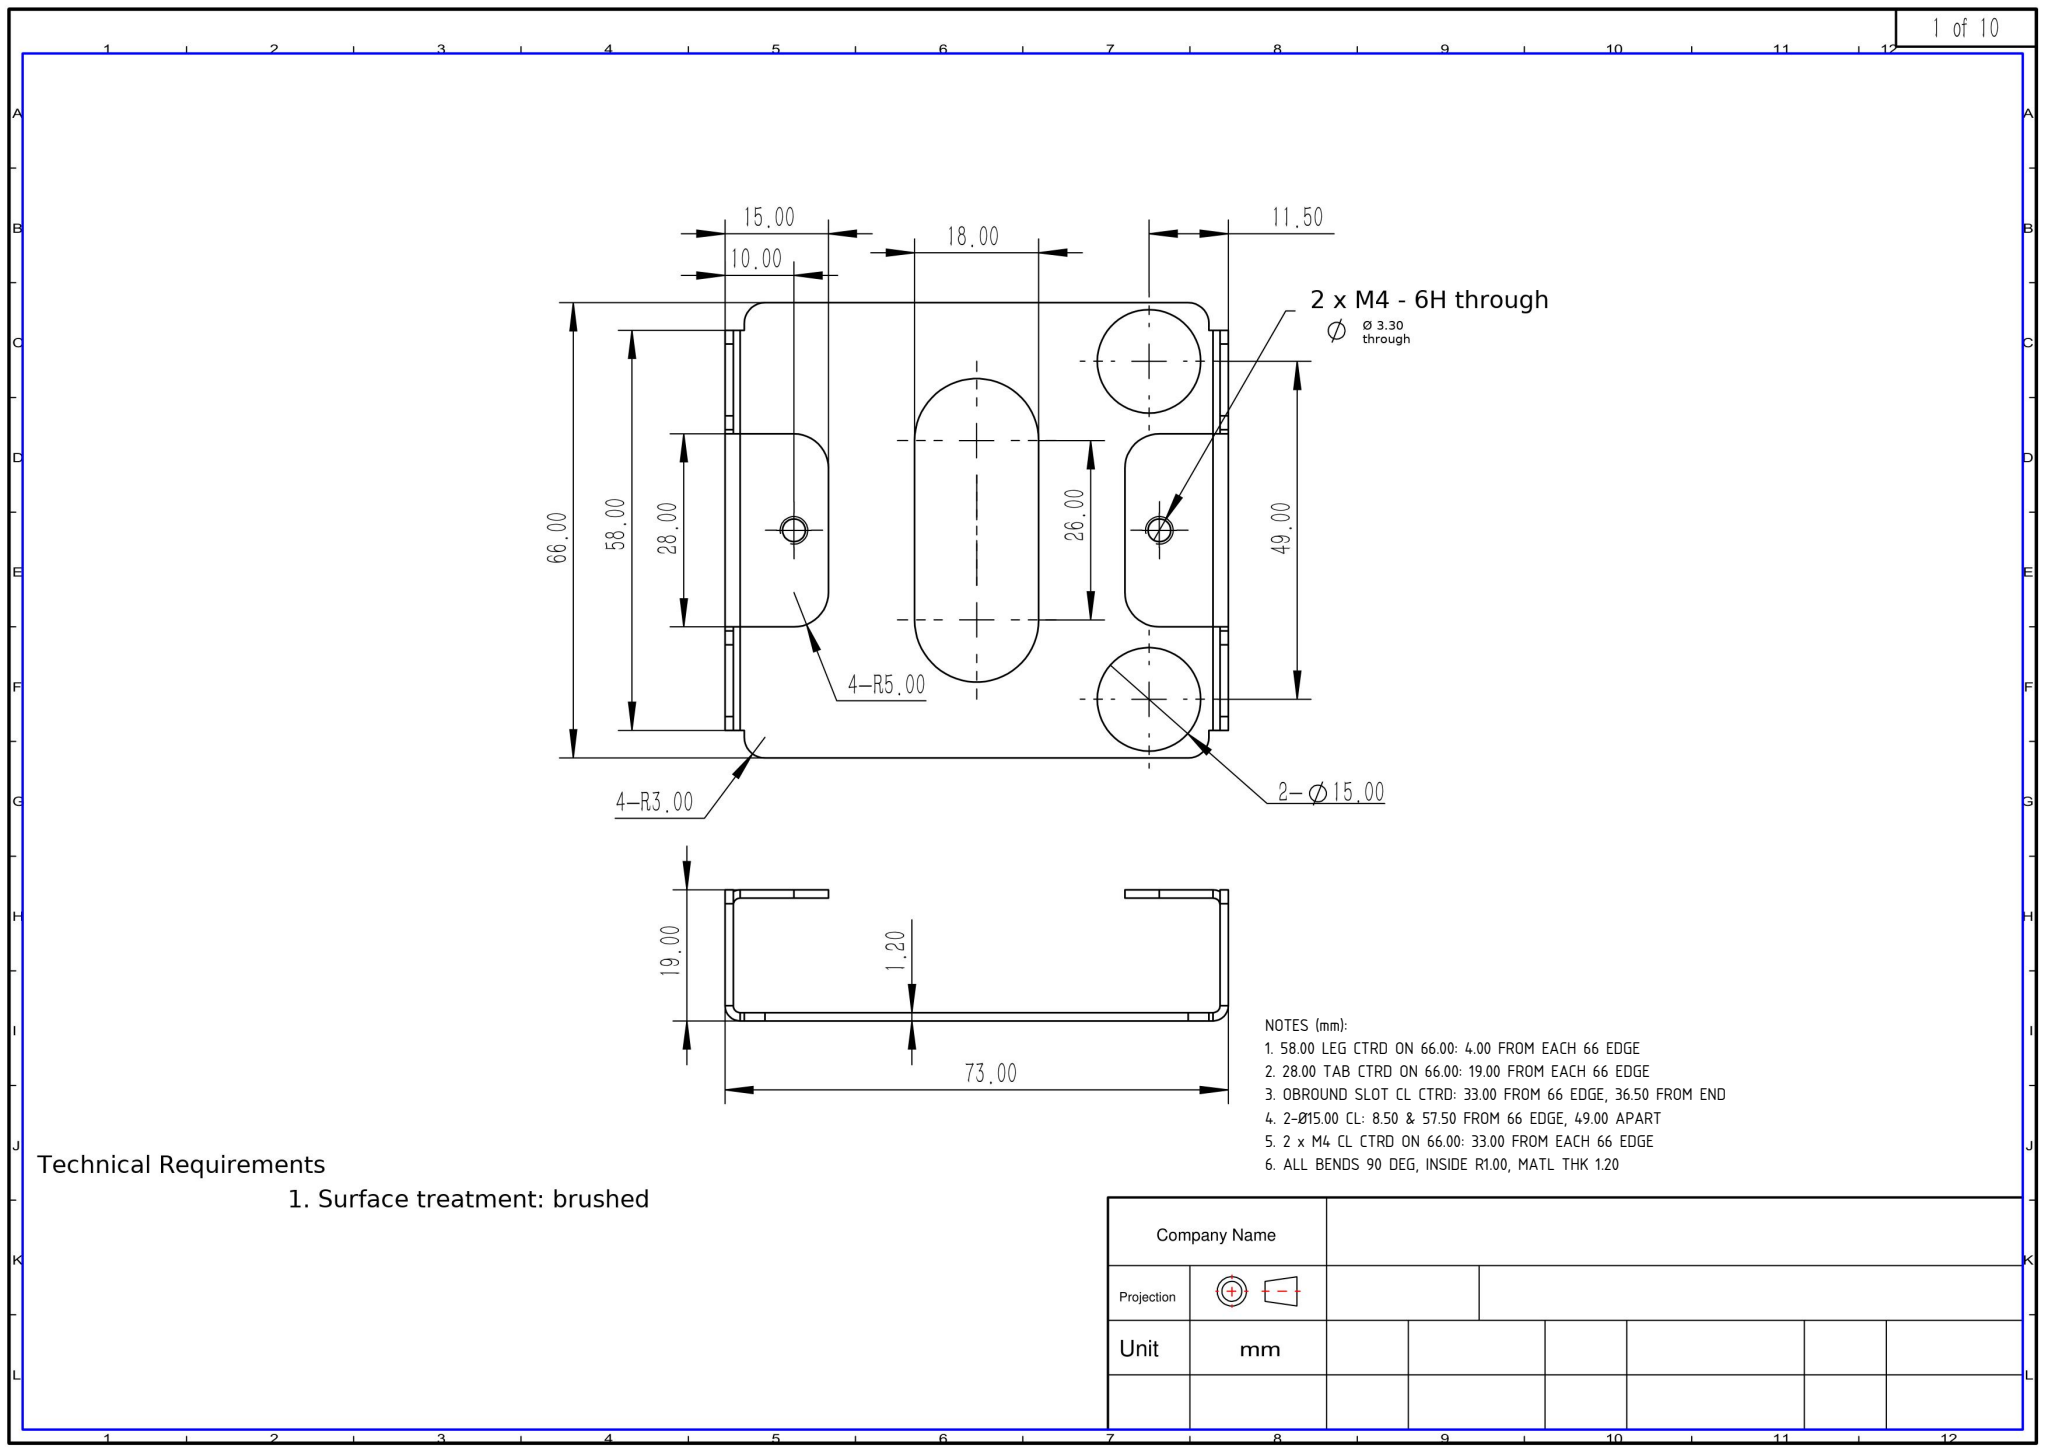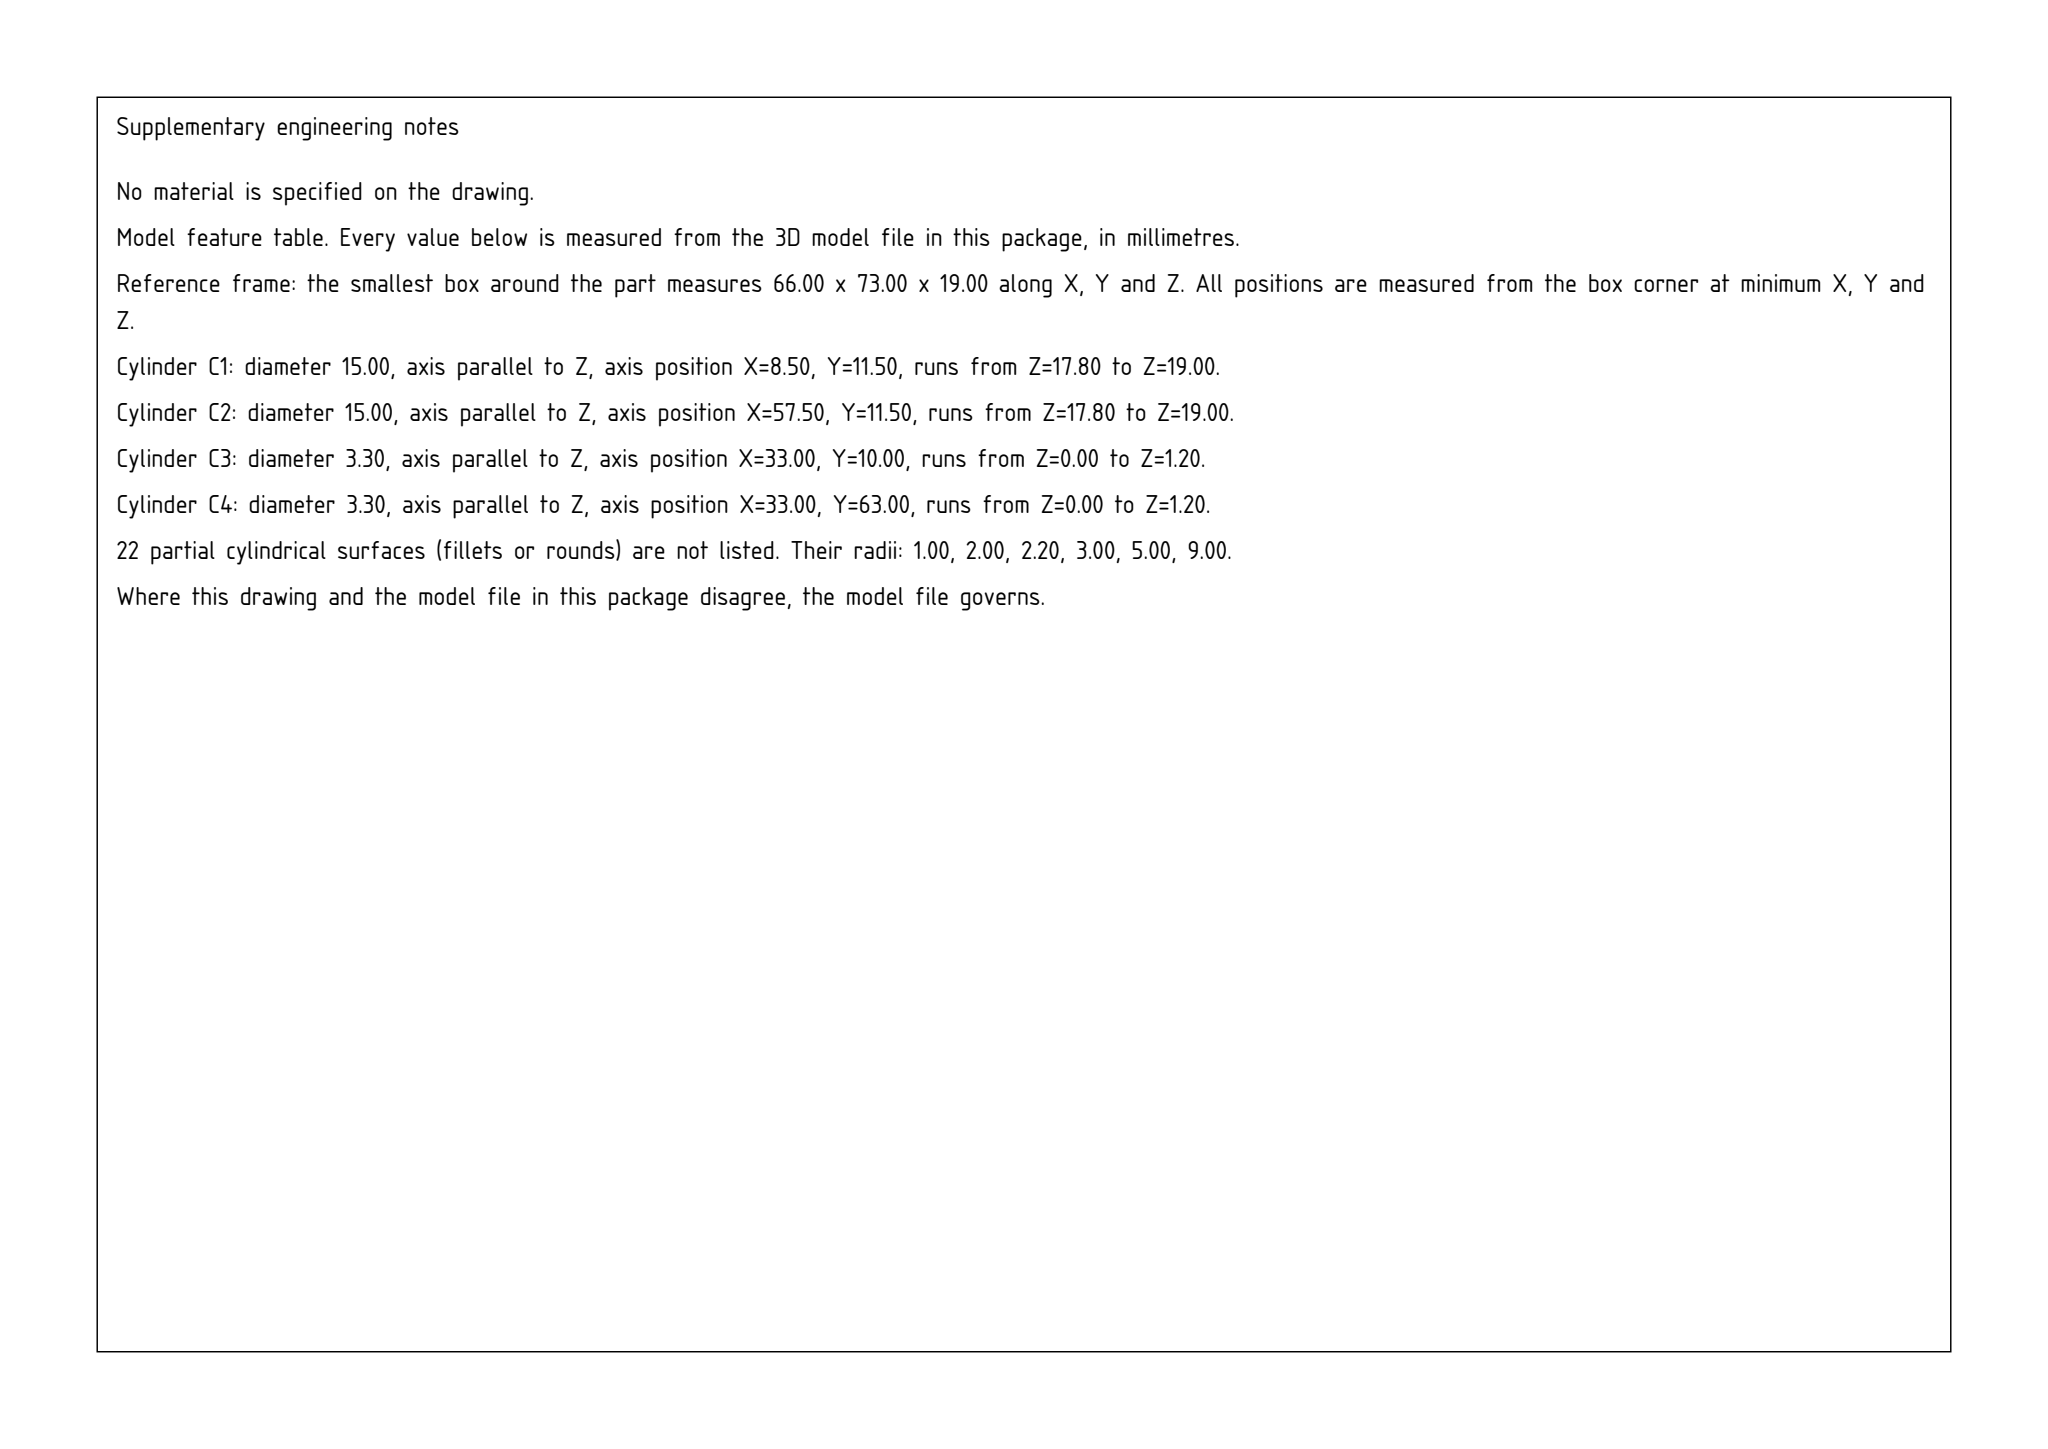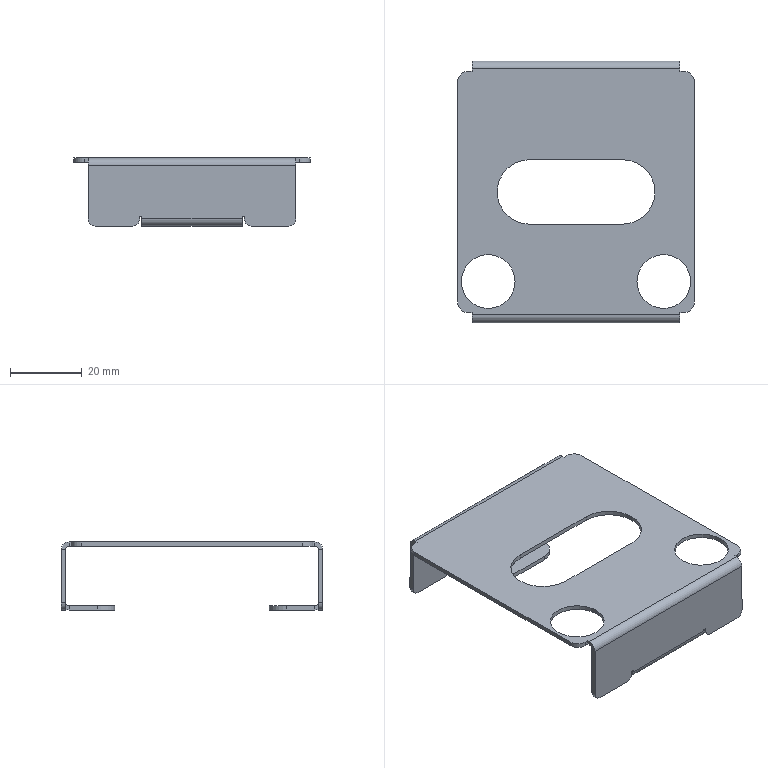Part | SolidWorks | mm | 1 solid | 91 faces | box 66 x 73 x 19 mm | volume 7628 mm3 | plane 56 | cylinder 35 | commonest cylinder face diameters 4 x8 3.3 x4 15 x4 4.4 x4 2 x4 10 x4 6 x4 18 x3
Drawing notes:
58.00 LEG CTRD ON 66.00: 4.00 FROM EACH 66 EDGE | from the solid: x planes at 4.0 & 62.0 (62-4=58), bend cyls len 58
28.00 TAB CTRD ON 66.00: 19.00 FROM EACH 66 EDGE | from the solid: x planes at 19.0 & 47.0 (47-19=28), bend cyls len 28
OBROUND SLOT CL CTRD: 33.00 FROM 66 EDGE, 36.50 FROM END | from the solid: Ø18 z-cyls at (20.0,36.5) & (46.0,36.5); midpt 33.0=66/2, 36.5=73/2
2-Ø15.00 CL: 8.50 & 57.50 FROM 66 EDGE, 49.00 APART | from the solid: Ø15 z-holes at x=8.5 & 57.5, y=11.5; 57.5-8.5=49.0
2 x M4 CL CTRD ON 66.00: 33.00 FROM EACH 66 EDGE | from the solid: Ø3.3 thru z-holes at x=33.0, y=10.0 & 63.0
ALL BENDS 90 DEG, INSIDE R1.00, MATL THK 1.20 | from the solid: bend cyls Ø2.0 inner / Ø4.4 outer, (4.4-2.0)/2=1.2 thk